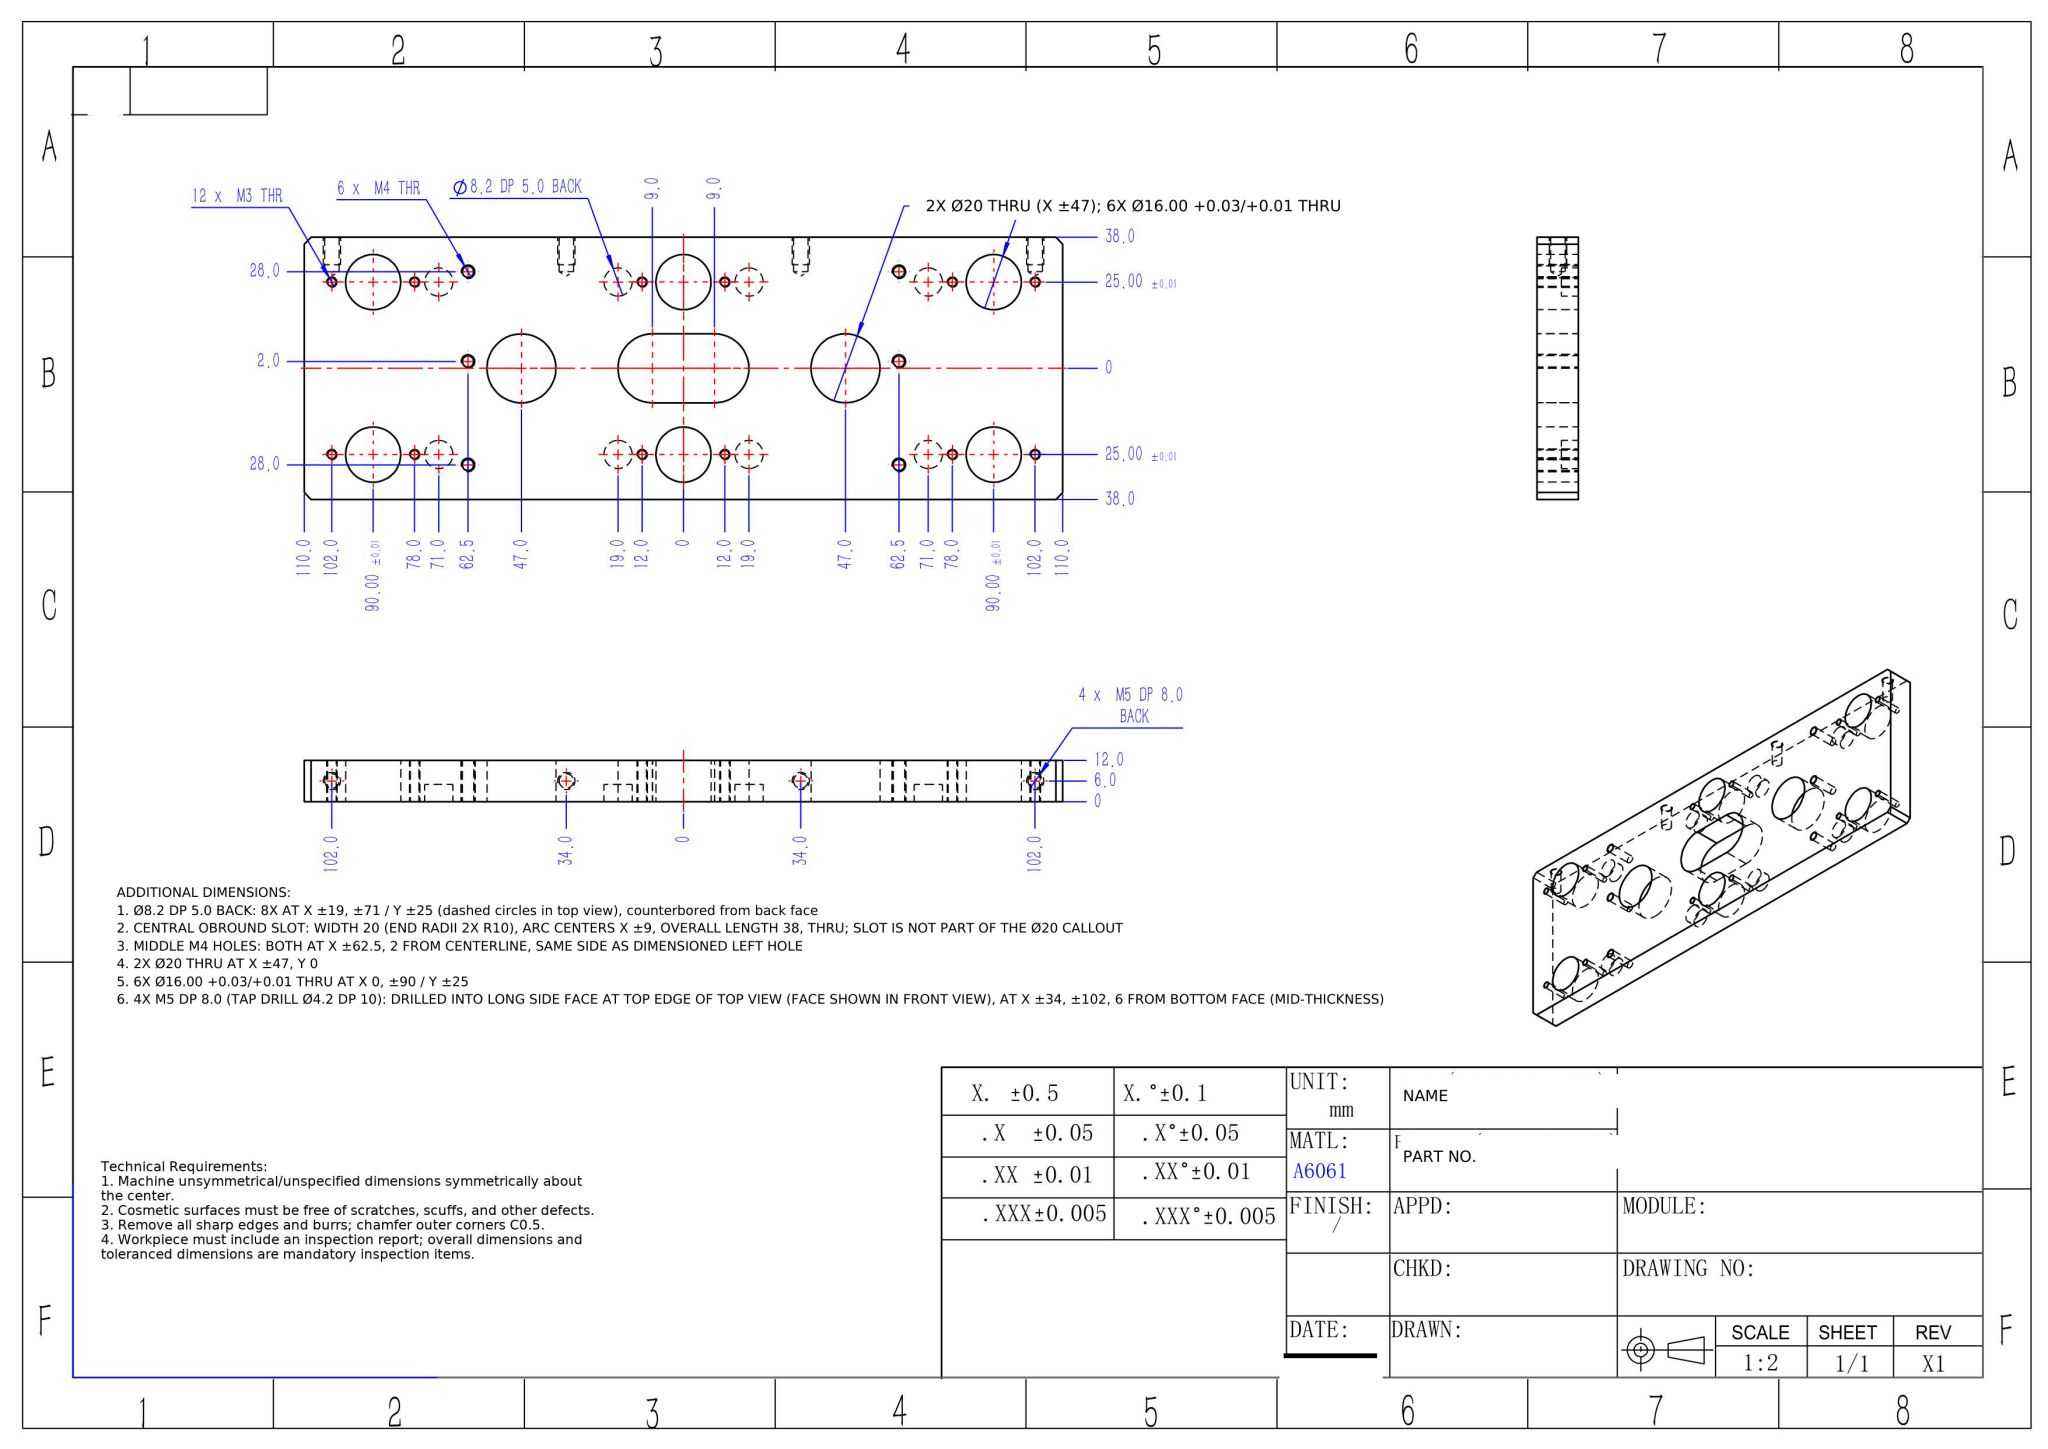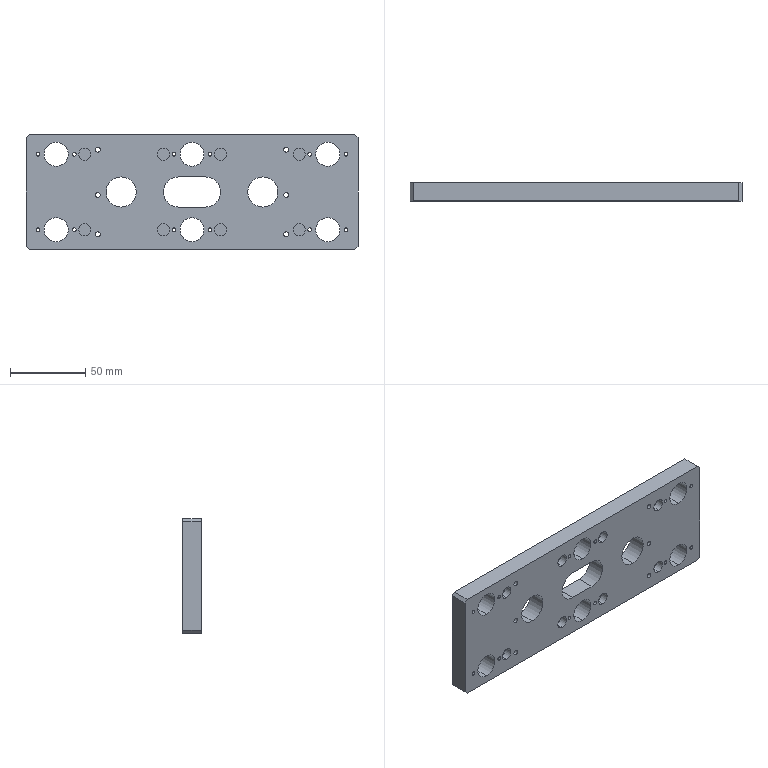Part | NX | mm | 1 solid | 106 faces | box 220 x 12 x 76 mm | volume 166425 mm3 | cylinder 78 | plane 20 | cone 8 | commonest cylinder face diameters 2.5 x24 8.2 x16 3.3 x12 16 x12 4.2 x8 20 x6